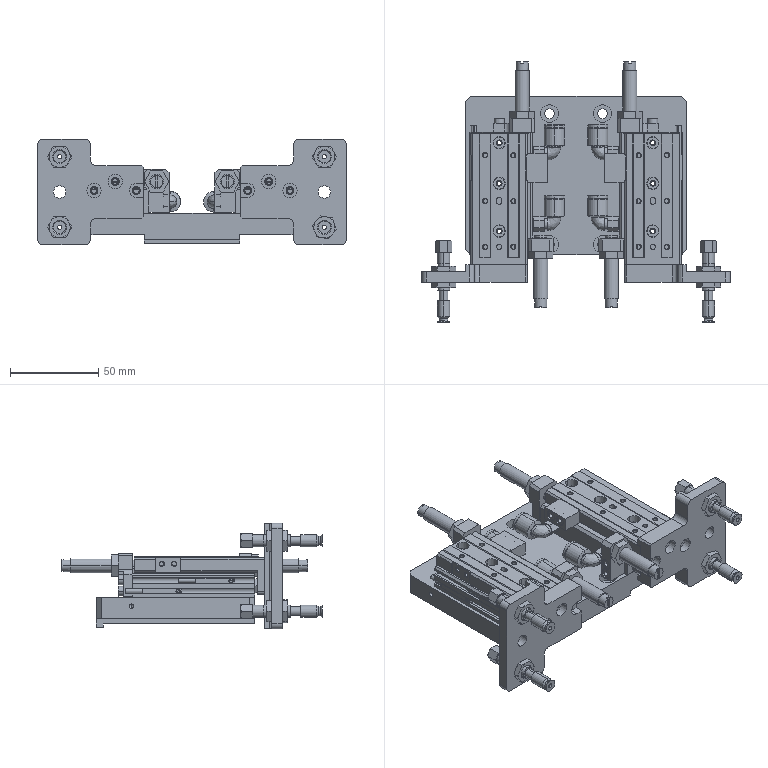Assembly | SolidWorks | mm | 37 component files | 37 solids | 1838 faces | box 175 x 147.3 x 60 mm | volume 317539 mm3 | plane 866 | cylinder 600 | cone 364 | spline 8 | commonest cylinder face diameters 2.459 x64 2.5 x40 5.5 x40 7 x40 6 x38 8 x36 3 x32 4 x32
Bill of materials:
KQ2L06-M5 | 4 |  | 90-degree elbow body: a large cylindrical barrel with a circumferential groove near its open end, joined by a curved tubular bend to a smaller straight branch carrying a hexagonal section and a stepped, chamfered cylindrical spigot.
MXQ8-30B-M9N_0_0_1_26 | 1 |  | Elongated prismatic block with a stepped (raised center) profile, three through-holes in a row along the top, and two semicircular longitudinal grooves running the full length of one side face.
MXQ8-30B-M9N_0_0_2_26 | 1 |  | Rectangular plate-like carriage block with a large L-shaped end portion; the top face has three large holes and several small holes, the end face has V-notched slots, and a thin rod with an end collar runs alongside, under the plate.
MXQ8-30B-M9N_0_0_3_25 | 1 |  | Plain rectangular block with a shallow vertical step or groove on one face and a small step near one top edge.
MXQ8-30B-M9N_0_0_4_20 | 1 |  | Shaft-and-bracket part: a stepped cylindrical shaft with a slotted end comes out of a hexagonal collar on an L-shaped block, and the block has a counterbored hole and two short cylindrical pins sticking out of its lower leg.
MXQ8-30B-M9N_0_0_5_16 | 1 |  | Stepped cylindrical shaft with a slotted end, passing through a hexagonal collar into a rectangular block with chamfered upper corners; a short shaft stub sticks out of the opposite side.
MXQ8-30B-M9N_0_0_6_4 | 1 |  | Long pin with a D-shaped cross-section (a cylinder with one large flat) over most of its length, stepping down to a smaller round cylindrical end.
MXQ8-30B-M9N_0_0_7_2 | 1 |  | Long pin with a D-shaped cross-section (a cylinder with one large flat) over most of its length, stepping down to a smaller round cylindrical end.
MXQ8L-30B-M9N_0_0_1_27 | 1 |  | Elongated prismatic block with a stepped (raised center) profile, three through-holes along the top, two semicircular longitudinal grooves on one side, and several round holes on the side and end faces.
MXQ8L-30B-M9N_0_0_2_27 | 1 |  | Rectangular plate-like carriage block with a large L-shaped end portion; the top face has three large holes and several small holes, the end face has V-notched slots, and a thin rod with an end collar runs alongside, under the plate.
MXQ8L-30B-M9N_0_0_3_26 | 1 |  | Rectangular block with two circular recesses on one long face, each holding a part with a hexagonal socket; there is a small step along one top edge.
MXQ8L-30B-M9N_0_0_4_21 | 1 |  | Shaft-and-bracket part: a stepped cylindrical shaft with a slotted end comes out of a hexagonal collar on an L-shaped block, and the block has a counterbored hole, a slot notch, and two short cylindrical pins on its lower leg.
MXQ8L-30B-M9N_0_0_5_17 | 1 |  | Stepped cylindrical pin or shaft: a longer, larger-diameter section with one flat along its length (D-shaped cross-section), then a shorter, smaller-diameter plain cylindrical section.
MXQ8L-30B-M9N_0_0_6_5 | 1 |  | Stepped cylindrical pin or shaft: a longer, larger-diameter section with one flat along its length (D-shaped cross-section), then a shorter, smaller-diameter plain cylindrical section.
MXQ8L-30B-M9N_0_0_7_3 | 1 |  | Combined body: a rectangular block with chamfered top corners, a hexagonal collar next to it, and a long stepped cylindrical shaft sticking out of the block. Near the shaft's free end there is a circumferential groove and a cross slot across the end face. Two round recessed features with hexagonal sockets sit side by side in a line on one face of the block. A short cylindrical stub sticks out from the opposite side of the block.
SAWH02-03329A0MountingBase | 1 | 6061 | Flat rectangular plate with small chamfers on all four corners. It has a pattern of through holes: four larger holes near the two long edges and ten smaller holes in a symmetric layout. A shallow raised pad or boss sticks out from the bottom face. One small hole is visible on a side edge face.
SAWH02-03330A0SuctionCupMountingBase | 1 | 6061 | T-shaped flat bracket plate. A wider rectangular section with rounded corners has three larger holes in a line. A narrower tab extends from it, with filleted inside corners and three smaller holes. The plate thickness is stepped, and the tab end has a notch or slot on its end face.
SAWH02-03342A0SuctionCupMountingBase(RightPart) | 1 | 6061 | T-shaped flat bracket plate. A wider rectangular section with rounded corners has three larger holes in a line. A narrower tab extends from it, with filleted inside corners, three smaller holes and small chamfers at its end corners. The plate thickness is stepped, and a slot is visible at the tab end.
Mates:
1. coincident | SAWH02-03330A0SuctionCupMountingBase-1 face at (-87.5, -60.5, 29.1) dir (0, -1, 0) | ZPT06UNK6_B5_A80214-1/ZPT2_8_B_NUT0214-2 face at (-69, -60.5, 9.1) dir (0, 1, 0)
2. concentric | SAWH02-03330A0SuctionCupMountingBase-1 face at (-75, -50.5, 9.1) dir (0, 1, 0) r 3.5 | ZPT06UNK6_B5_A80214-1/ZPT06U6_B5_B_BUFFER0214-1 face at (-75, -71, 9.1) dir (0, 1, 0) r 3.458
3. concentric | SAWH02-03330A0SuctionCupMountingBase-1 face at (-75, -50.5, 49.1) dir (0, 1, 0) r 3.5 | ZPT06UNK6_B5_A80214-2/ZPT06U6_B5_B_BUFFER0214-1 face at (-75, -71, 49.1) dir (0, 1, 0) r 3.458
4. coincident | SAWH02-03330A0SuctionCupMountingBase-1 face at (-87.5, -60.5, 29.1) dir (0, -1, 0) | ZPT06UNK6_B5_A80214-2/ZPT2_8_B_NUT0214-2 face at (-69, -60.5, 49.1) dir (0, 1, 0)
5. concentric | SAWH02-03329A0MountingBase-1 face at (43.5, 18.5, 17) dir (0, 0, 1) r 1.25 | MXQ8-30B-M9N_0_0_MXQ8-30B-M9N_0_0-2/MXQ8-30B-M9N_0_0_1_26-1 face at (43.5, 18.5, 21.189) dir (0, 0, -1) r 1.621
6. concentric | SAWH02-03329A0MountingBase-1 face at (43.5, -4.5, 17) dir (0, 0, 1) r 1.25 | MXQ8-30B-M9N_0_0_MXQ8-30B-M9N_0_0-2/MXQ8-30B-M9N_0_0_1_26-1 face at (43.5, -4.5, 21.189) dir (0, 0, -1) r 1.621
7. coincident | SAWH02-03329A0MountingBase-1 face at (0, 0, 17) dir (0, 0, 1) | MXQ8-30B-M9N_0_0_MXQ8-30B-M9N_0_0-2/MXQ8-30B-M9N_0_0_1_26-1 face at (60.5, 24.5, 17) dir (0, 0, -1)
8. coincident | MXQ8-30B-M9N_0_0_MXQ8-30B-M9N_0_0-2/MXQ8-30B-M9N_0_0_2_26-1 face at (43.5, -52.5, 17) dir (0, -1, 0) | SAWH02-03342A0SuctionCupMountingBase(RightPart)-2 face at (59.5, -52.5, 18.5) dir (0, 1, 0)
9. coincident | MXQ8-30B-M9N_0_0_MXQ8-30B-M9N_0_0-2/MXQ8-30B-M9N_0_0_2_26-1 face at (59.5, 23.5, 38.7) dir (1, 0, 0) | SAWH02-03342A0SuctionCupMountingBase(RightPart)-2 face at (59.5, -52.5, 38.2) dir (-1, 0, 0)
10. coincident | MXQ8-30B-M9N_0_0_MXQ8-30B-M9N_0_0-2/MXQ8-30B-M9N_0_0_2_26-1 face at (28.5, 23.5, 39.7) dir (0, 0, 1) | SAWH02-03342A0SuctionCupMountingBase(RightPart)-2 face at (58, -52.5, 39.7) dir (0, 0, -1)
11. coincident | SAWH02-03342A0SuctionCupMountingBase(RightPart)-2 face at (87.5, -60.5, 29.1) dir (0, -1, 0) | ZPT06UNK6_B5_A80214-3/ZPT2_8_B_NUT0214-2 face at (81, -60.5, 49.1) dir (0, 1, 0)
12. concentric | SAWH02-03342A0SuctionCupMountingBase(RightPart)-2 face at (75, -50.5, 9.1) dir (0, 1, 0) r 3.5 | ZPT06UNK6_B5_A80214-4/ZPT06U6_B5_B_BUFFER0214-1 face at (75, -71, 9.1) dir (0, 1, 0) r 3.458
13. coincident | SAWH02-03342A0SuctionCupMountingBase(RightPart)-2 face at (87.5, -60.5, 29.1) dir (0, -1, 0) | ZPT06UNK6_B5_A80214-4/ZPT2_8_B_NUT0214-2 face at (77.116, -60.5, 3.485) dir (0, 1, 0)
14. concentric | SAWH02-03329A0MountingBase-1 face at (-43.5, 18.5, 17) dir (0, 0, 1) r 1.25 | MXQ8L-30B-M9N_0_0_MXQ8L-30B-M9N_0_0-1/MXQ8L-30B-M9N_0_0_1_27-1 face at (-43.5, 18.5, 21.189) dir (0, 0, -1) r 1.621
15. concentric | SAWH02-03329A0MountingBase-1 face at (-43.5, -4.5, 17) dir (0, 0, 1) r 1.25 | MXQ8L-30B-M9N_0_0_MXQ8L-30B-M9N_0_0-1/MXQ8L-30B-M9N_0_0_1_27-1 face at (-43.5, -4.5, 21.189) dir (0, 0, -1) r 1.621
16. coincident | SAWH02-03329A0MountingBase-1 face at (0, 0, 17) dir (0, 0, 1) | MXQ8L-30B-M9N_0_0_MXQ8L-30B-M9N_0_0-1/MXQ8L-30B-M9N_0_0_1_27-1 face at (-24.5, 24.5, 17) dir (0, 0, -1)
17. coincident | SAWH02-03330A0SuctionCupMountingBase-1 face at (-59.5, -52.5, 39.7) dir (0, 1, 0) | MXQ8L-30B-M9N_0_0_MXQ8L-30B-M9N_0_0-1/MXQ8L-30B-M9N_0_0_2_27-1 face at (-43.5, -52.5, 17) dir (0, -1, 0)
18. coincident | SAWH02-03330A0SuctionCupMountingBase-1 face at (-59.5, -52.5, 20) dir (1, 0, 0) | MXQ8L-30B-M9N_0_0_MXQ8L-30B-M9N_0_0-1/MXQ8L-30B-M9N_0_0_2_27-1 face at (-59.5, 23.5, 32) dir (-1, 0, 0)
19. coincident | SAWH02-03330A0SuctionCupMountingBase-1 face at (-58, -52.5, 39.7) dir (0, 0, -1) | MXQ8L-30B-M9N_0_0_MXQ8L-30B-M9N_0_0-1/MXQ8L-30B-M9N_0_0_2_27-1 face at (-58.5, 23.5, 39.7) dir (0, 0, 1)
20. concentric | SAWH02-03342A0SuctionCupMountingBase(RightPart)-2 face at (75, -50.5, 49.1) dir (0, 1, 0) r 3.5 | ZPT06UNK6_B5_A80214-3/ZPT06U6_B5_B_BUFFER0214-1 face at (75, -71, 49.1) dir (0, 1, 0) r 3.458
21. concentric | MXQ8-30B-M9N_0_0_1_26-1 face at (-16.784, 6.5, 12) dir (1, 0, 0) r 2.067 | KQ2L06-M5-1 face at (-17.75, 6.5, 12) dir (-1, 0, 0) r 2.5
22. coincident | MXQ8-30B-M9N_0_0_1_26-1 face at (-19, 0, 0) dir (-1, 0, 0) | KQ2L06-M5-1 face at (-19, 9.08, 12) dir (1, 0, 0)
23. concentric | MXQ8-30B-M9N_0_0_1_26-1 face at (-16.784, 6.5, 52) dir (1, 0, 0) r 2.067 | KQ2L06-M5-2 face at (-17.75, 6.5, 52) dir (-1, 0, 0) r 2.5
24. coincident | MXQ8-30B-M9N_0_0_1_26-1 face at (-19, 0, 0) dir (-1, 0, 0) | KQ2L06-M5-2 face at (-19, 9.08, 52) dir (1, 0, 0)
25. concentric | MXQ8L-30B-M9N_0_0_1_27-1 edge at (15, 6.5, 12) dir (1, 0, 0) r 2.067 | KQ2L06-M5-1 face at (17.75, 6.5, 12) dir (1, 0, 0) r 2.5
26. coincident | MXQ8L-30B-M9N_0_0_1_27-1 face at (19, 12.439, 0) dir (1, 0, 0) | KQ2L06-M5-1 face at (19, 3.921, 11.954) dir (-1, 0, 0)
27. concentric | MXQ8L-30B-M9N_0_0_1_27-1 face at (16.784, 6.5, 52) dir (1, 0, 0) r 2.067 | KQ2L06-M5-2 face at (17.75, 6.5, 52) dir (1, 0, 0) r 2.5
28. coincident | MXQ8L-30B-M9N_0_0_1_27-1 face at (19, 12.439, 0) dir (1, 0, 0) | KQ2L06-M5-2 face at (19, 3.921, 51.954) dir (-1, 0, 0)
29. distance | ZPT2_8_B_NUT0214-1 plane at (0, 30, 0) dir (0, -1, 0) | ZPT06U6_B5_B_BUFFER0214-1 plane at (0, 25.5, 0) dir (0, 1, 0)
30. coincident | ZPT06U6_B5_B_BUFFER0214-1 axis at (0, 50, 0) dir (0, -1, 0) | ZPT2_8_B_NUT0214-1 axis at (0, -20, 0) dir (0, 1, 0)
31. distance | ZPT2_8_B_NUT0214-2 plane at (0, 21, 0) dir (0, -1, 0) | ZPT06U6_B5_B_BUFFER0214-1 plane at (0, 25.5, 0) dir (0, 1, 0)
32. coincident | ZPT06U6_B5_B_BUFFER0214-1 axis at (0, 50, 0) dir (0, -1, 0) | ZPT2_8_B_NUT0214-2 axis at (0, -29, 0) dir (0, 1, 0)